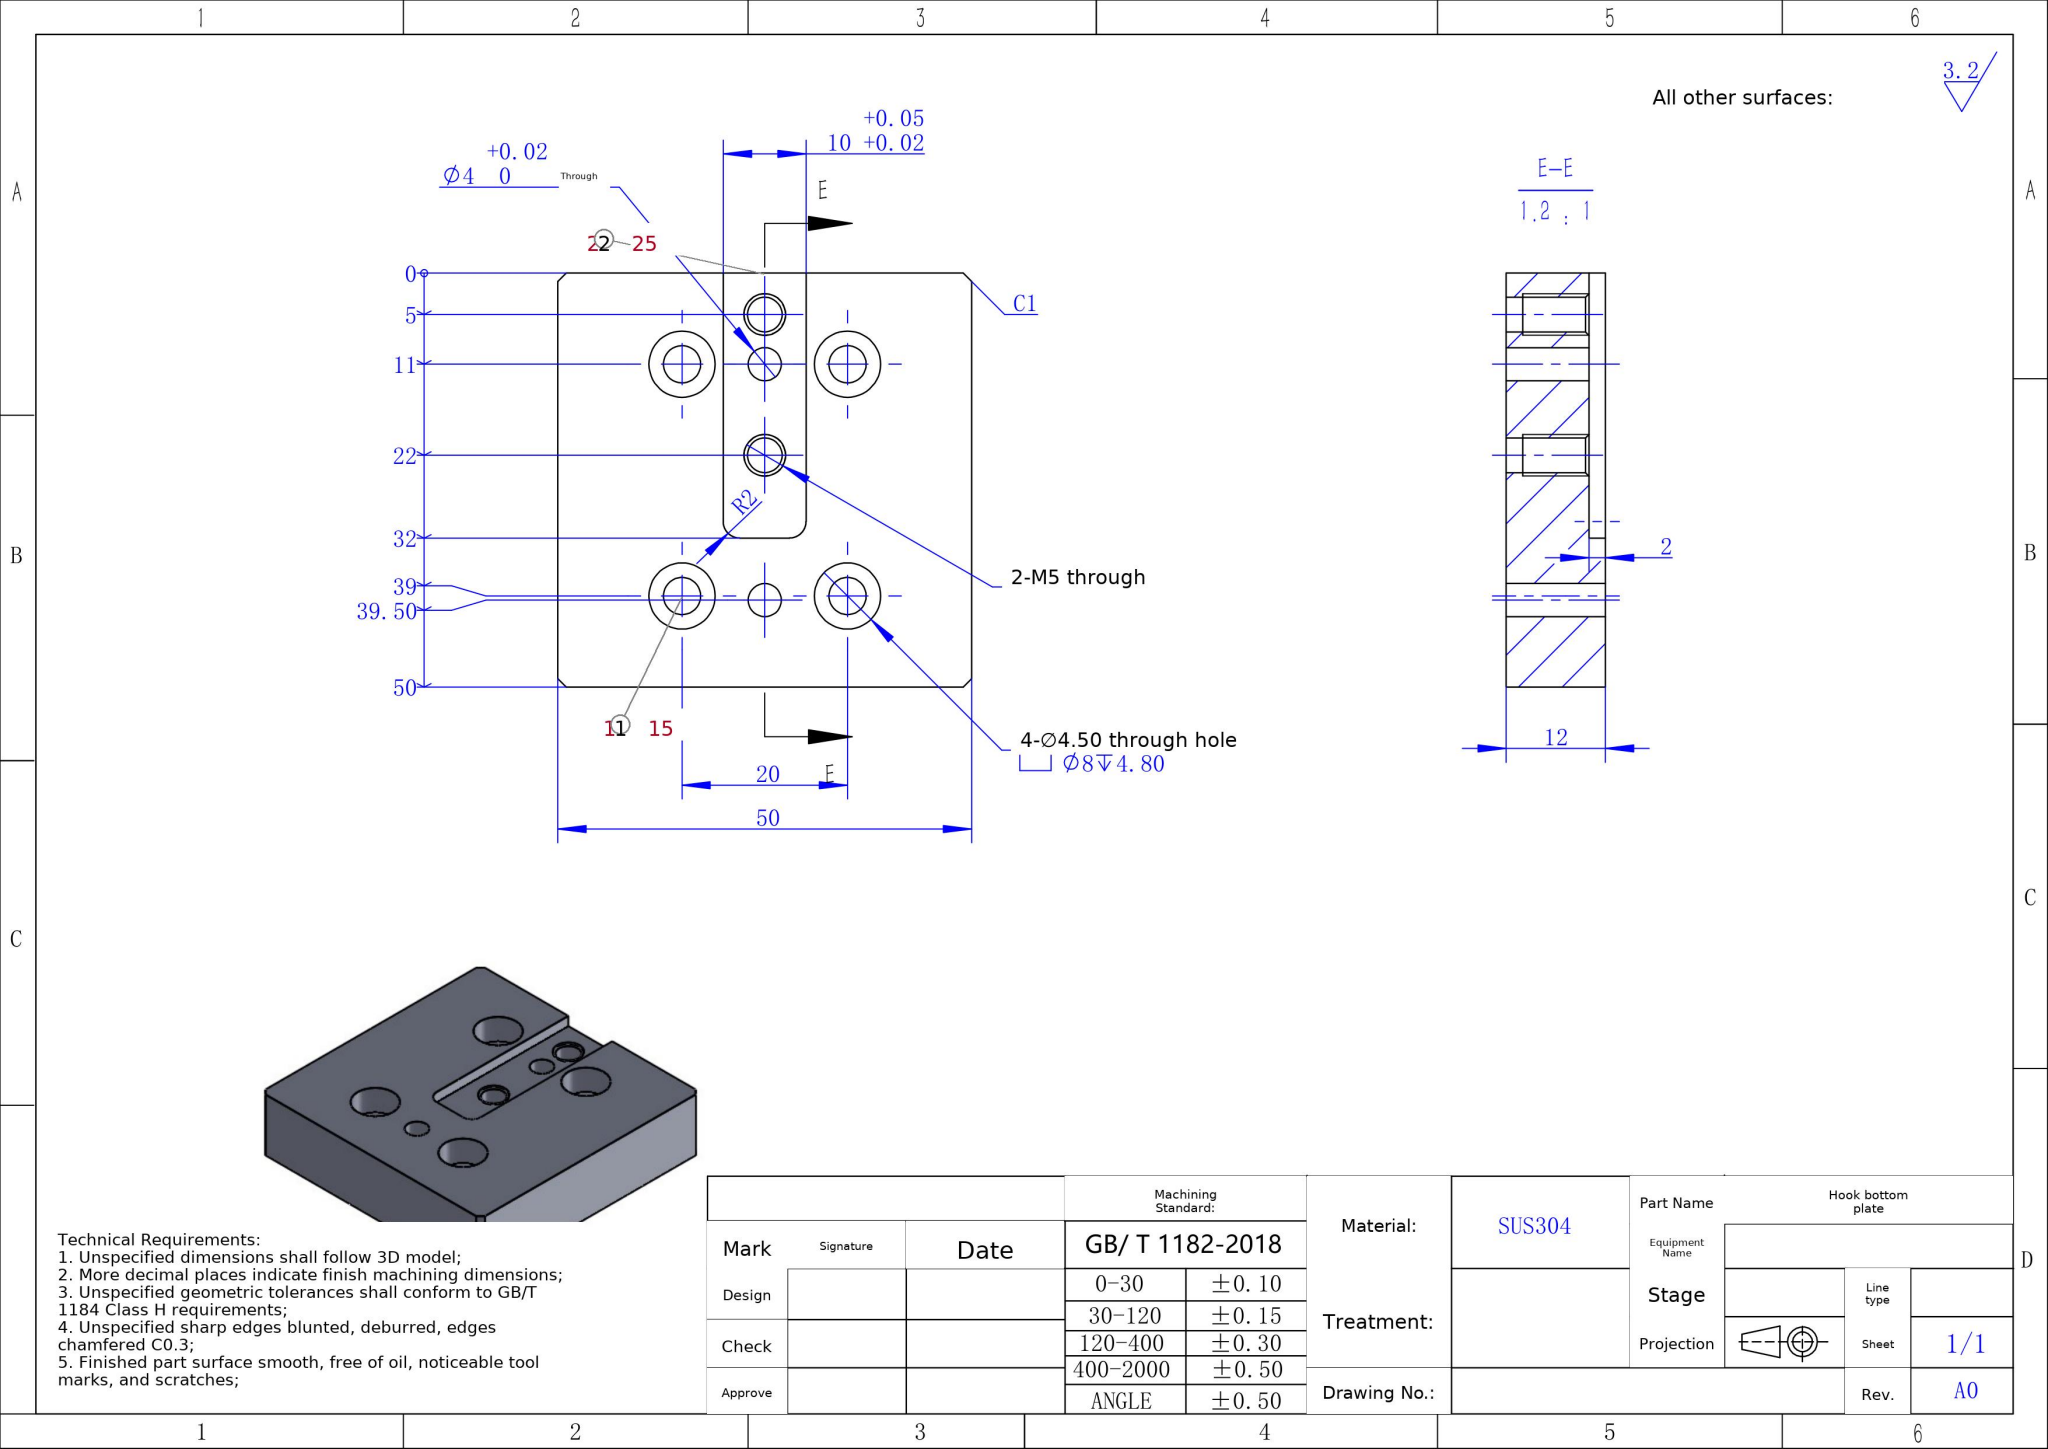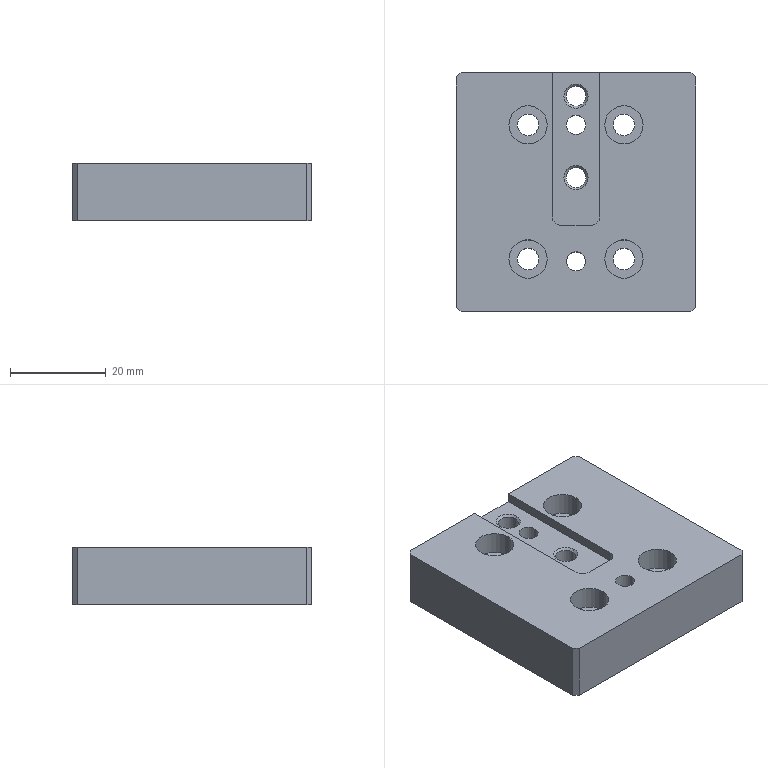Part | SolidWorks | mm | material SUS304 | 1 solid | 48 faces | box 50 x 50 x 12 mm | volume 27360 mm3 | cylinder 26 | plane 18 | cone 4 | commonest cylinder face diameters 8 x8 4.5 x8 4 x6 4.2 x4